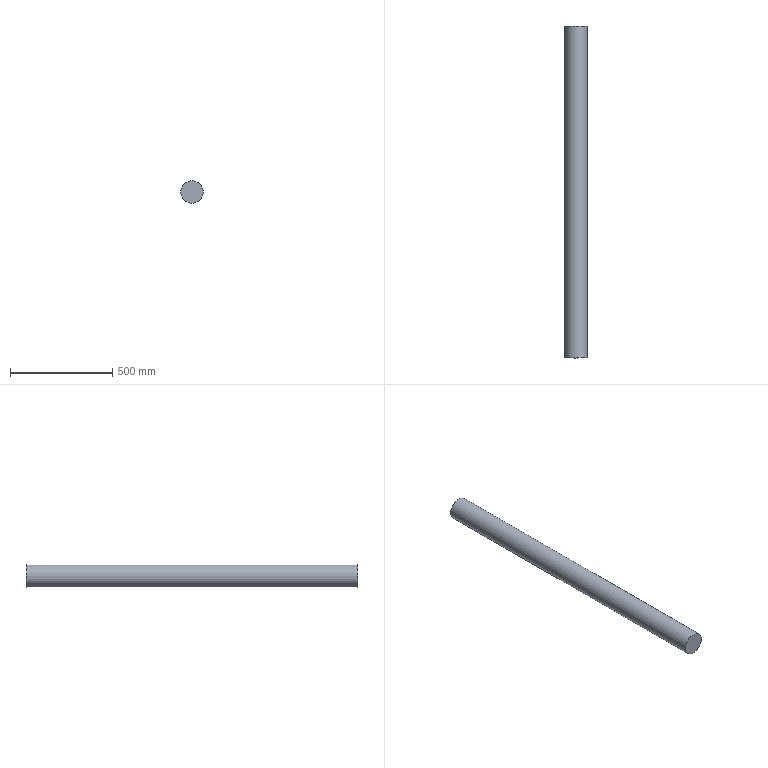Component | NX | AXIAL1 | 1 solid | 3 faces | box 110 x 1620 x 110 mm | volume 15395375 mm3 | plane 2 | cylinder 1 | commonest cylinder face diameters 110 x1
STEP:
#1=CARTESIAN_POINT('',(0.,0.,0.));
#2=DIRECTION('',(0.,0.,1.));
#3=DIRECTION('',(1.,0.,0.));
#4=AXIS2_PLACEMENT_3D('',#1,#2,#3);
#5=CARTESIAN_POINT('',(812.906,1710.,705.841));
#6=VERTEX_POINT('',#5);
#7=CARTESIAN_POINT('',(757.906,1710.,705.841));
#8=DIRECTION('',(0.,-1.,0.));
#9=DIRECTION('',(1.,0.,0.));
#10=AXIS2_PLACEMENT_3D('',#7,#8,#9);
#11=CIRCLE('',#10,55.);
#12=CARTESIAN_POINT('',(757.906,1710.,705.841));
#13=DIRECTION('',(0.,-1.,0.));
#14=DIRECTION('',(0.,0.,-1.));
#15=AXIS2_PLACEMENT_3D('',#12,#13,#14);
#16=CYLINDRICAL_SURFACE('',#15,55.);
#17=CARTESIAN_POINT('',(1.571,0.));
#18=DIRECTION('',(1.,0.));
#19=VECTOR('',#18,1.);
#20=LINE('',#17,#19);
#21=(GEOMETRIC_REPRESENTATION_CONTEXT(2)PARAMETRIC_REPRESENTATION_CONTEXT()REPRESENTATION_CONTEXT('',''));
#22=DEFINITIONAL_REPRESENTATION('',(#20),#21);
#23=PCURVE('',#16,#22);
#24=CARTESIAN_POINT('',(757.906,1710.,705.841));
#25=DIRECTION('',(0.,-1.,0.));
#26=DIRECTION('',(0.,0.,-1.));
#27=AXIS2_PLACEMENT_3D('',#24,#25,#26);
#28=PLANE('',#27);
#29=CARTESIAN_POINT('',(0.,0.));
#30=DIRECTION('',(0.,1.));
#31=AXIS2_PLACEMENT_2D('',#29,#30);
#32=CIRCLE('',#31,55.);
#33=(GEOMETRIC_REPRESENTATION_CONTEXT(2)PARAMETRIC_REPRESENTATION_CONTEXT()REPRESENTATION_CONTEXT('',''));
#34=DEFINITIONAL_REPRESENTATION('',(#32),#33);
#35=PCURVE('',#28,#34);
#36=SURFACE_CURVE('',#11,(#23,#35),.PCURVE_S1.);
#37=EDGE_CURVE('',#6,#6,#36,.T.);
#38=ORIENTED_EDGE('',*,*,#37,.T.);
#39=CARTESIAN_POINT('',(812.906,90.,705.841));
#40=VERTEX_POINT('',#39);
#41=CARTESIAN_POINT('',(812.906,1710.,705.841));
#42=CARTESIAN_POINT('',(812.906,90.,705.841));
#43=B_SPLINE_CURVE_WITH_KNOTS('',1,(#41,#42),.UNSPECIFIED.,.F.,.F.,(2,2),(0.,1620.),.PIECEWISE_BEZIER_KNOTS.);
#44=CARTESIAN_POINT('',(7.854,0.));
#45=DIRECTION('',(0.,1.));
#46=VECTOR('',#45,1.);
#47=LINE('',#44,#46);
#48=(GEOMETRIC_REPRESENTATION_CONTEXT(2)PARAMETRIC_REPRESENTATION_CONTEXT()REPRESENTATION_CONTEXT('',''));
#49=DEFINITIONAL_REPRESENTATION('',(#47),#48);
#50=PCURVE('',#16,#49);
#51=CARTESIAN_POINT('',(1.571,0.));
#52=DIRECTION('',(0.,1.));
#53=VECTOR('',#52,1.);
#54=LINE('',#51,#53);
#55=(GEOMETRIC_REPRESENTATION_CONTEXT(2)PARAMETRIC_REPRESENTATION_CONTEXT()REPRESENTATION_CONTEXT('',''));
#56=DEFINITIONAL_REPRESENTATION('',(#54),#55);
#57=PCURVE('',#16,#56);
#58=SEAM_CURVE('',#43,(#50,#57),.PCURVE_S1.);
#59=EDGE_CURVE('',#6,#40,#58,.T.);
#60=ORIENTED_EDGE('',*,*,#59,.T.);
#61=CARTESIAN_POINT('',(757.906,90.,705.841));
#62=DIRECTION('',(0.,-1.,0.));
#63=DIRECTION('',(1.,0.,0.));
#64=AXIS2_PLACEMENT_3D('',#61,#62,#63);
#65=CIRCLE('',#64,55.);
#66=CARTESIAN_POINT('',(1.571,1620.));
#67=DIRECTION('',(1.,0.));
#68=VECTOR('',#67,1.);
#69=LINE('',#66,#68);
#70=(GEOMETRIC_REPRESENTATION_CONTEXT(2)PARAMETRIC_REPRESENTATION_CONTEXT()REPRESENTATION_CONTEXT('',''));
#71=DEFINITIONAL_REPRESENTATION('',(#69),#70);
#72=PCURVE('',#16,#71);
#73=CARTESIAN_POINT('',(757.906,90.,705.841));
#74=DIRECTION('',(0.,-1.,0.));
#75=DIRECTION('',(0.,0.,-1.));
#76=AXIS2_PLACEMENT_3D('',#73,#74,#75);
#77=PLANE('',#76);
#78=CARTESIAN_POINT('',(0.,0.));
#79=DIRECTION('',(0.,1.));
#80=AXIS2_PLACEMENT_2D('',#78,#79);
#81=CIRCLE('',#80,55.);
#82=(GEOMETRIC_REPRESENTATION_CONTEXT(2)PARAMETRIC_REPRESENTATION_CONTEXT()REPRESENTATION_CONTEXT('',''));
#83=DEFINITIONAL_REPRESENTATION('',(#81),#82);
#84=PCURVE('',#77,#83);
#85=SURFACE_CURVE('',#65,(#72,#84),.PCURVE_S1.);
#86=EDGE_CURVE('',#40,#40,#85,.T.);
#87=ORIENTED_EDGE('',*,*,#86,.F.);
#88=ORIENTED_EDGE('',*,*,#59,.F.);
#89=EDGE_LOOP('',(#38,#60,#87,#88));
#90=FACE_BOUND('',#89,.T.);
#91=ADVANCED_FACE('',(#90),#16,.T.);
#92=ORIENTED_EDGE('',*,*,#37,.F.);
#93=EDGE_LOOP('',(#92));
#94=FACE_BOUND('',#93,.T.);
#95=ADVANCED_FACE('',(#94),#28,.F.);
#96=ORIENTED_EDGE('',*,*,#86,.T.);
#97=EDGE_LOOP('',(#96));
#98=FACE_BOUND('',#97,.T.);
#99=ADVANCED_FACE('',(#98),#77,.T.);
#100=CLOSED_SHELL('',(#91,#95,#99));
#101=MANIFOLD_SOLID_BREP('',#100);
#102=(LENGTH_UNIT()NAMED_UNIT(*)SI_UNIT(.MILLI.,.METRE.));
#103=UNCERTAINTY_MEASURE_WITH_UNIT(LENGTH_MEASURE(0.00001),#102,'','');
#104=(NAMED_UNIT(*)PLANE_ANGLE_UNIT()SI_UNIT($,.RADIAN.));
#105=(NAMED_UNIT(*)SI_UNIT($,.STERADIAN.)SOLID_ANGLE_UNIT());
#106=(GEOMETRIC_REPRESENTATION_CONTEXT(3)GLOBAL_UNCERTAINTY_ASSIGNED_CONTEXT((#103))GLOBAL_UNIT_ASSIGNED_CONTEXT((#102,#104,#105))REPRESENTATION_CONTEXT('',''));
#107=ADVANCED_BREP_SHAPE_REPRESENTATION('',(#4,#101),#106);